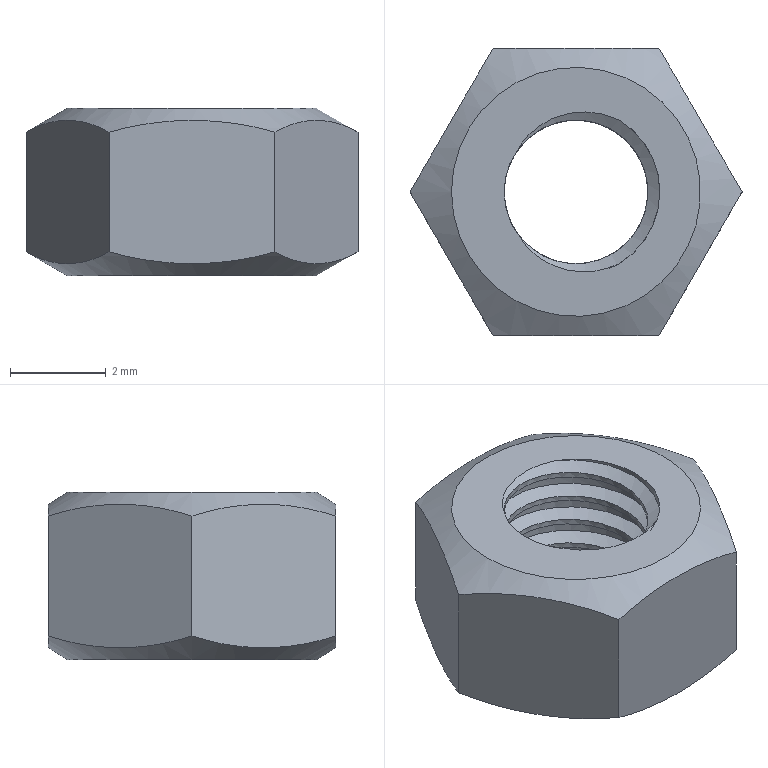Component | NX | NUT_M3 | 1 solid | 14 faces | volume 76 mm3 | plane 8 | cylinder 2 | spline 2 | cone 2 | commonest cylinder face diameters 3 x1 3.5 x1